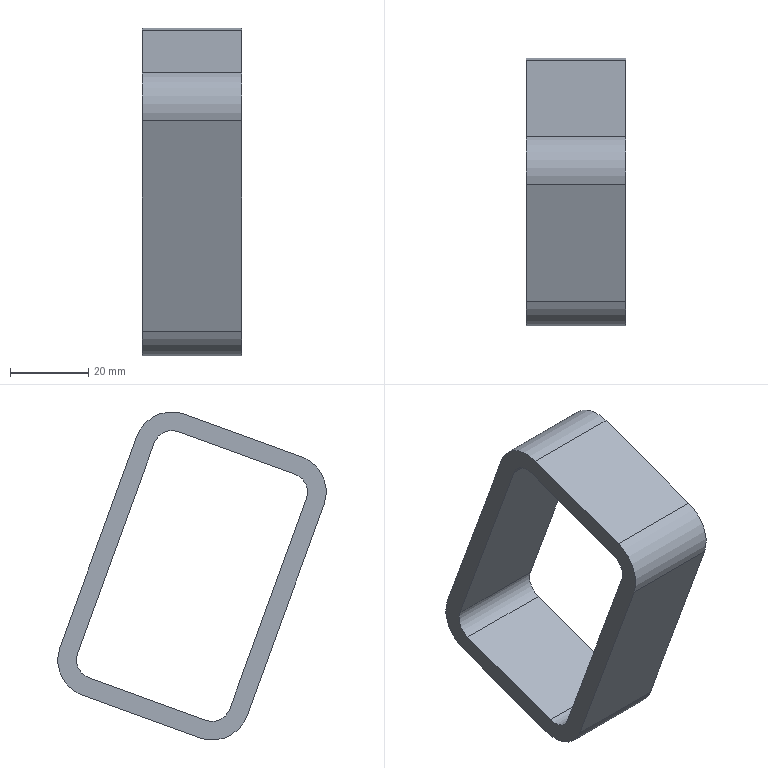Component | SolidWorks | rectangular tube_iso-69 | 1 solid | 18 faces | box 25.4 x 68.44 x 83.61 mm | volume 26938 mm3 | plane 10 | cylinder 8 | commonest cylinder face diameters 19.05 x4 9.525 x4
STEP:
#1=COLOUR_RGB('',0.7922,0.8196,0.9333);
#2=FILL_AREA_STYLE_COLOUR('',#1);
#3=FILL_AREA_STYLE('',(#2));
#4=SURFACE_STYLE_FILL_AREA(#3);
#5=SURFACE_SIDE_STYLE('',(#4));
#6=SURFACE_STYLE_USAGE(.BOTH.,#5);
#7=PRESENTATION_STYLE_ASSIGNMENT((#6));
#8=CARTESIAN_POINT('',(1.827,-40.871,5.613));
#9=VERTEX_POINT('',#8);
#10=CARTESIAN_POINT('',(1.827,-40.391,5.389));
#11=VERTEX_POINT('',#10);
#12=CARTESIAN_POINT('',(1.827,-40.519,5.741));
#13=DIRECTION('',(1.,-0.,0.));
#14=DIRECTION('',(0.,-0.9397,-0.3421));
#15=AXIS2_PLACEMENT_3D('',#12,#13,#14);
#16=CIRCLE('',#15,0.375);
#17=EDGE_CURVE('',#9,#11,#16,.T.);
#18=ORIENTED_EDGE('',*,*,#17,.T.);
#19=CARTESIAN_POINT('',(1.827,-39.216,5.817));
#20=VERTEX_POINT('',#19);
#21=CARTESIAN_POINT('',(1.827,-40.391,5.389));
#22=DIRECTION('',(0.,0.9397,0.3421));
#23=VECTOR('',#22,39.37);
#24=LINE('',#21,#23);
#25=EDGE_CURVE('',#11,#20,#24,.T.);
#26=ORIENTED_EDGE('',*,*,#25,.T.);
#27=CARTESIAN_POINT('',(1.827,-38.992,6.297));
#28=VERTEX_POINT('',#27);
#29=CARTESIAN_POINT('',(1.827,-39.344,6.169));
#30=DIRECTION('',(1.,-0.,0.));
#31=DIRECTION('',(0.,-0.9397,-0.3421));
#32=AXIS2_PLACEMENT_3D('',#29,#30,#31);
#33=CIRCLE('',#32,0.375);
#34=EDGE_CURVE('',#20,#28,#33,.T.);
#35=ORIENTED_EDGE('',*,*,#34,.T.);
#36=CARTESIAN_POINT('',(1.827,-39.762,8.412));
#37=VERTEX_POINT('',#36);
#38=CARTESIAN_POINT('',(1.827,-39.762,8.412));
#39=DIRECTION('',(-0.,-0.3421,0.9397));
#40=VECTOR('',#39,39.37);
#41=LINE('',#38,#40);
#42=EDGE_CURVE('',#28,#37,#41,.T.);
#43=ORIENTED_EDGE('',*,*,#42,.T.);
#44=CARTESIAN_POINT('',(1.827,-40.242,8.636));
#45=VERTEX_POINT('',#44);
#46=CARTESIAN_POINT('',(1.827,-40.114,8.283));
#47=DIRECTION('',(1.,-0.,0.));
#48=DIRECTION('',(0.,-0.9397,-0.3421));
#49=AXIS2_PLACEMENT_3D('',#46,#47,#48);
#50=CIRCLE('',#49,0.375);
#51=EDGE_CURVE('',#37,#45,#50,.T.);
#52=ORIENTED_EDGE('',*,*,#51,.T.);
#53=CARTESIAN_POINT('',(1.827,-41.417,8.208));
#54=VERTEX_POINT('',#53);
#55=CARTESIAN_POINT('',(1.827,-40.242,8.636));
#56=DIRECTION('',(-0.,-0.9397,-0.3421));
#57=VECTOR('',#56,39.37);
#58=LINE('',#55,#57);
#59=EDGE_CURVE('',#45,#54,#58,.T.);
#60=ORIENTED_EDGE('',*,*,#59,.T.);
#61=CARTESIAN_POINT('',(1.827,-41.641,7.727));
#62=VERTEX_POINT('',#61);
#63=CARTESIAN_POINT('',(1.827,-41.289,7.856));
#64=DIRECTION('',(1.,-0.,0.));
#65=DIRECTION('',(0.,-0.9397,-0.3421));
#66=AXIS2_PLACEMENT_3D('',#63,#64,#65);
#67=CIRCLE('',#66,0.375);
#68=EDGE_CURVE('',#54,#62,#67,.T.);
#69=ORIENTED_EDGE('',*,*,#68,.T.);
#70=CARTESIAN_POINT('',(1.827,-40.871,5.613));
#71=DIRECTION('',(0.,0.3421,-0.9397));
#72=VECTOR('',#71,39.37);
#73=LINE('',#70,#72);
#74=EDGE_CURVE('',#62,#9,#73,.T.);
#75=ORIENTED_EDGE('',*,*,#74,.T.);
#76=EDGE_LOOP('',(#18,#26,#35,#43,#52,#60,#69,#75));
#77=FACE_OUTER_BOUND('',#76,.T.);
#78=CARTESIAN_POINT('',(1.827,-39.168,6.233));
#79=VERTEX_POINT('',#78);
#80=CARTESIAN_POINT('',(1.827,-39.938,8.347));
#81=VERTEX_POINT('',#80);
#82=CARTESIAN_POINT('',(1.827,-39.938,8.347));
#83=DIRECTION('',(-0.,-0.3421,0.9397));
#84=VECTOR('',#83,39.37);
#85=LINE('',#82,#84);
#86=EDGE_CURVE('',#79,#81,#85,.T.);
#87=ORIENTED_EDGE('',*,*,#86,.F.);
#88=CARTESIAN_POINT('',(1.827,-39.28,5.993));
#89=VERTEX_POINT('',#88);
#90=CARTESIAN_POINT('',(1.827,-39.344,6.169));
#91=DIRECTION('',(1.,-0.,0.));
#92=DIRECTION('',(0.,-0.9397,-0.3421));
#93=AXIS2_PLACEMENT_3D('',#90,#91,#92);
#94=CIRCLE('',#93,0.1875);
#95=EDGE_CURVE('',#89,#79,#94,.T.);
#96=ORIENTED_EDGE('',*,*,#95,.F.);
#97=CARTESIAN_POINT('',(1.827,-40.455,5.565));
#98=VERTEX_POINT('',#97);
#99=CARTESIAN_POINT('',(1.827,-40.455,5.565));
#100=DIRECTION('',(0.,0.9397,0.3421));
#101=VECTOR('',#100,39.37);
#102=LINE('',#99,#101);
#103=EDGE_CURVE('',#98,#89,#102,.T.);
#104=ORIENTED_EDGE('',*,*,#103,.F.);
#105=CARTESIAN_POINT('',(1.827,-40.695,5.677));
#106=VERTEX_POINT('',#105);
#107=CARTESIAN_POINT('',(1.827,-40.519,5.741));
#108=DIRECTION('',(1.,-0.,0.));
#109=DIRECTION('',(0.,-0.9397,-0.3421));
#110=AXIS2_PLACEMENT_3D('',#107,#108,#109);
#111=CIRCLE('',#110,0.1875);
#112=EDGE_CURVE('',#106,#98,#111,.T.);
#113=ORIENTED_EDGE('',*,*,#112,.F.);
#114=CARTESIAN_POINT('',(1.827,-41.465,7.791));
#115=VERTEX_POINT('',#114);
#116=CARTESIAN_POINT('',(1.827,-40.695,5.677));
#117=DIRECTION('',(0.,0.3421,-0.9397));
#118=VECTOR('',#117,39.37);
#119=LINE('',#116,#118);
#120=EDGE_CURVE('',#115,#106,#119,.T.);
#121=ORIENTED_EDGE('',*,*,#120,.F.);
#122=CARTESIAN_POINT('',(1.827,-41.353,8.032));
#123=VERTEX_POINT('',#122);
#124=CARTESIAN_POINT('',(1.827,-41.289,7.856));
#125=DIRECTION('',(1.,-0.,0.));
#126=DIRECTION('',(0.,-0.9397,-0.3421));
#127=AXIS2_PLACEMENT_3D('',#124,#125,#126);
#128=CIRCLE('',#127,0.1875);
#129=EDGE_CURVE('',#123,#115,#128,.T.);
#130=ORIENTED_EDGE('',*,*,#129,.F.);
#131=CARTESIAN_POINT('',(1.827,-40.178,8.459));
#132=VERTEX_POINT('',#131);
#133=CARTESIAN_POINT('',(1.827,-40.178,8.459));
#134=DIRECTION('',(-0.,-0.9397,-0.3421));
#135=VECTOR('',#134,39.37);
#136=LINE('',#133,#135);
#137=EDGE_CURVE('',#132,#123,#136,.T.);
#138=ORIENTED_EDGE('',*,*,#137,.F.);
#139=CARTESIAN_POINT('',(1.827,-40.114,8.283));
#140=DIRECTION('',(1.,-0.,0.));
#141=DIRECTION('',(0.,-0.9397,-0.3421));
#142=AXIS2_PLACEMENT_3D('',#139,#140,#141);
#143=CIRCLE('',#142,0.1875);
#144=EDGE_CURVE('',#81,#132,#143,.T.);
#145=ORIENTED_EDGE('',*,*,#144,.F.);
#146=EDGE_LOOP('',(#87,#96,#104,#113,#121,#130,#138,#145));
#147=FACE_BOUND('',#146,.T.);
#148=CARTESIAN_POINT('',(1.827,-40.519,5.741));
#149=DIRECTION('',(1.,-0.,0.));
#150=DIRECTION('',(-0.,-0.9397,-0.3421));
#151=AXIS2_PLACEMENT_3D('',#148,#149,#150);
#152=PLANE('',#151);
#153=ADVANCED_FACE('',(#77,#147),#152,.T.);
#154=CARTESIAN_POINT('',(0.8268,-40.871,5.613));
#155=VERTEX_POINT('',#154);
#156=CARTESIAN_POINT('',(0.8268,-40.391,5.389));
#157=VERTEX_POINT('',#156);
#158=CARTESIAN_POINT('',(0.8268,-40.519,5.741));
#159=DIRECTION('',(1.,-0.,0.));
#160=DIRECTION('',(0.,-0.9397,-0.3421));
#161=AXIS2_PLACEMENT_3D('',#158,#159,#160);
#162=CIRCLE('',#161,0.375);
#163=EDGE_CURVE('',#155,#157,#162,.T.);
#164=ORIENTED_EDGE('',*,*,#163,.F.);
#165=CARTESIAN_POINT('',(0.8268,-41.641,7.727));
#166=VERTEX_POINT('',#165);
#167=CARTESIAN_POINT('',(0.8268,-40.871,5.613));
#168=DIRECTION('',(0.,0.3421,-0.9397));
#169=VECTOR('',#168,39.37);
#170=LINE('',#167,#169);
#171=EDGE_CURVE('',#166,#155,#170,.T.);
#172=ORIENTED_EDGE('',*,*,#171,.F.);
#173=CARTESIAN_POINT('',(0.8268,-41.417,8.208));
#174=VERTEX_POINT('',#173);
#175=CARTESIAN_POINT('',(0.8268,-41.289,7.856));
#176=DIRECTION('',(1.,-0.,0.));
#177=DIRECTION('',(0.,-0.9397,-0.3421));
#178=AXIS2_PLACEMENT_3D('',#175,#176,#177);
#179=CIRCLE('',#178,0.375);
#180=EDGE_CURVE('',#174,#166,#179,.T.);
#181=ORIENTED_EDGE('',*,*,#180,.F.);
#182=CARTESIAN_POINT('',(0.8268,-40.242,8.636));
#183=VERTEX_POINT('',#182);
#184=CARTESIAN_POINT('',(0.8268,-40.242,8.636));
#185=DIRECTION('',(-0.,-0.9397,-0.3421));
#186=VECTOR('',#185,39.37);
#187=LINE('',#184,#186);
#188=EDGE_CURVE('',#183,#174,#187,.T.);
#189=ORIENTED_EDGE('',*,*,#188,.F.);
#190=CARTESIAN_POINT('',(0.8268,-39.762,8.412));
#191=VERTEX_POINT('',#190);
#192=CARTESIAN_POINT('',(0.8268,-40.114,8.283));
#193=DIRECTION('',(1.,-0.,0.));
#194=DIRECTION('',(0.,-0.9397,-0.3421));
#195=AXIS2_PLACEMENT_3D('',#192,#193,#194);
#196=CIRCLE('',#195,0.375);
#197=EDGE_CURVE('',#191,#183,#196,.T.);
#198=ORIENTED_EDGE('',*,*,#197,.F.);
#199=CARTESIAN_POINT('',(0.8268,-38.992,6.297));
#200=VERTEX_POINT('',#199);
#201=CARTESIAN_POINT('',(0.8268,-39.762,8.412));
#202=DIRECTION('',(-0.,-0.3421,0.9397));
#203=VECTOR('',#202,39.37);
#204=LINE('',#201,#203);
#205=EDGE_CURVE('',#200,#191,#204,.T.);
#206=ORIENTED_EDGE('',*,*,#205,.F.);
#207=CARTESIAN_POINT('',(0.8268,-39.216,5.817));
#208=VERTEX_POINT('',#207);
#209=CARTESIAN_POINT('',(0.8268,-39.344,6.169));
#210=DIRECTION('',(1.,-0.,0.));
#211=DIRECTION('',(0.,-0.9397,-0.3421));
#212=AXIS2_PLACEMENT_3D('',#209,#210,#211);
#213=CIRCLE('',#212,0.375);
#214=EDGE_CURVE('',#208,#200,#213,.T.);
#215=ORIENTED_EDGE('',*,*,#214,.F.);
#216=CARTESIAN_POINT('',(0.8268,-40.391,5.389));
#217=DIRECTION('',(0.,0.9397,0.3421));
#218=VECTOR('',#217,39.37);
#219=LINE('',#216,#218);
#220=EDGE_CURVE('',#157,#208,#219,.T.);
#221=ORIENTED_EDGE('',*,*,#220,.F.);
#222=EDGE_LOOP('',(#164,#172,#181,#189,#198,#206,#215,#221));
#223=FACE_OUTER_BOUND('',#222,.T.);
#224=CARTESIAN_POINT('',(0.8268,-39.28,5.993));
#225=VERTEX_POINT('',#224);
#226=CARTESIAN_POINT('',(0.8268,-39.168,6.233));
#227=VERTEX_POINT('',#226);
#228=CARTESIAN_POINT('',(0.8268,-39.344,6.169));
#229=DIRECTION('',(1.,-0.,0.));
#230=DIRECTION('',(0.,-0.9397,-0.3421));
#231=AXIS2_PLACEMENT_3D('',#228,#229,#230);
#232=CIRCLE('',#231,0.1875);
#233=EDGE_CURVE('',#225,#227,#232,.T.);
#234=ORIENTED_EDGE('',*,*,#233,.T.);
#235=CARTESIAN_POINT('',(0.8268,-39.938,8.347));
#236=VERTEX_POINT('',#235);
#237=CARTESIAN_POINT('',(0.8268,-39.938,8.347));
#238=DIRECTION('',(-0.,-0.3421,0.9397));
#239=VECTOR('',#238,39.37);
#240=LINE('',#237,#239);
#241=EDGE_CURVE('',#227,#236,#240,.T.);
#242=ORIENTED_EDGE('',*,*,#241,.T.);
#243=CARTESIAN_POINT('',(0.8268,-40.178,8.459));
#244=VERTEX_POINT('',#243);
#245=CARTESIAN_POINT('',(0.8268,-40.114,8.283));
#246=DIRECTION('',(1.,-0.,0.));
#247=DIRECTION('',(0.,-0.9397,-0.3421));
#248=AXIS2_PLACEMENT_3D('',#245,#246,#247);
#249=CIRCLE('',#248,0.1875);
#250=EDGE_CURVE('',#236,#244,#249,.T.);
#251=ORIENTED_EDGE('',*,*,#250,.T.);
#252=CARTESIAN_POINT('',(0.8268,-41.353,8.032));
#253=VERTEX_POINT('',#252);
#254=CARTESIAN_POINT('',(0.8268,-40.178,8.459));
#255=DIRECTION('',(-0.,-0.9397,-0.3421));
#256=VECTOR('',#255,39.37);
#257=LINE('',#254,#256);
#258=EDGE_CURVE('',#244,#253,#257,.T.);
#259=ORIENTED_EDGE('',*,*,#258,.T.);
#260=CARTESIAN_POINT('',(0.8268,-41.465,7.791));
#261=VERTEX_POINT('',#260);
#262=CARTESIAN_POINT('',(0.8268,-41.289,7.856));
#263=DIRECTION('',(1.,-0.,0.));
#264=DIRECTION('',(0.,-0.9397,-0.3421));
#265=AXIS2_PLACEMENT_3D('',#262,#263,#264);
#266=CIRCLE('',#265,0.1875);
#267=EDGE_CURVE('',#253,#261,#266,.T.);
#268=ORIENTED_EDGE('',*,*,#267,.T.);
#269=CARTESIAN_POINT('',(0.8268,-40.695,5.677));
#270=VERTEX_POINT('',#269);
#271=CARTESIAN_POINT('',(0.8268,-40.695,5.677));
#272=DIRECTION('',(0.,0.3421,-0.9397));
#273=VECTOR('',#272,39.37);
#274=LINE('',#271,#273);
#275=EDGE_CURVE('',#261,#270,#274,.T.);
#276=ORIENTED_EDGE('',*,*,#275,.T.);
#277=CARTESIAN_POINT('',(0.8268,-40.455,5.565));
#278=VERTEX_POINT('',#277);
#279=CARTESIAN_POINT('',(0.8268,-40.519,5.741));
#280=DIRECTION('',(1.,-0.,0.));
#281=DIRECTION('',(0.,-0.9397,-0.3421));
#282=AXIS2_PLACEMENT_3D('',#279,#280,#281);
#283=CIRCLE('',#282,0.1875);
#284=EDGE_CURVE('',#270,#278,#283,.T.);
#285=ORIENTED_EDGE('',*,*,#284,.T.);
#286=CARTESIAN_POINT('',(0.8268,-40.455,5.565));
#287=DIRECTION('',(0.,0.9397,0.3421));
#288=VECTOR('',#287,39.37);
#289=LINE('',#286,#288);
#290=EDGE_CURVE('',#278,#225,#289,.T.);
#291=ORIENTED_EDGE('',*,*,#290,.T.);
#292=EDGE_LOOP('',(#234,#242,#251,#259,#268,#276,#285,#291));
#293=FACE_BOUND('',#292,.T.);
#294=CARTESIAN_POINT('',(0.8268,-40.519,5.741));
#295=DIRECTION('',(1.,-0.,0.));
#296=DIRECTION('',(-0.,-0.9397,-0.3421));
#297=AXIS2_PLACEMENT_3D('',#294,#295,#296);
#298=PLANE('',#297);
#299=ADVANCED_FACE('',(#223,#293),#298,.F.);
#300=ORIENTED_EDGE('',*,*,#163,.T.);
#301=CARTESIAN_POINT('',(1.827,-40.391,5.389));
#302=DIRECTION('',(-1.,0.,-0.));
#303=VECTOR('',#302,39.37);
#304=LINE('',#301,#303);
#305=EDGE_CURVE('',#11,#157,#304,.T.);
#306=ORIENTED_EDGE('',*,*,#305,.F.);
#307=ORIENTED_EDGE('',*,*,#17,.F.);
#308=CARTESIAN_POINT('',(1.827,-40.871,5.613));
#309=DIRECTION('',(-1.,0.,-0.));
#310=VECTOR('',#309,39.37);
#311=LINE('',#308,#310);
#312=EDGE_CURVE('',#9,#155,#311,.T.);
#313=ORIENTED_EDGE('',*,*,#312,.T.);
#314=EDGE_LOOP('',(#300,#306,#307,#313));
#315=FACE_OUTER_BOUND('',#314,.T.);
#316=CARTESIAN_POINT('',(1.827,-40.519,5.741));
#317=DIRECTION('',(-1.,0.,-0.));
#318=DIRECTION('',(0.,0.9397,0.3421));
#319=AXIS2_PLACEMENT_3D('',#316,#317,#318);
#320=CYLINDRICAL_SURFACE('',#319,0.375);
#321=ADVANCED_FACE('',(#315),#320,.T.);
#322=ORIENTED_EDGE('',*,*,#220,.T.);
#323=CARTESIAN_POINT('',(1.827,-39.216,5.817));
#324=DIRECTION('',(-1.,0.,-0.));
#325=VECTOR('',#324,39.37);
#326=LINE('',#323,#325);
#327=EDGE_CURVE('',#20,#208,#326,.T.);
#328=ORIENTED_EDGE('',*,*,#327,.F.);
#329=ORIENTED_EDGE('',*,*,#25,.F.);
#330=ORIENTED_EDGE('',*,*,#305,.T.);
#331=EDGE_LOOP('',(#322,#328,#329,#330));
#332=FACE_OUTER_BOUND('',#331,.T.);
#333=CARTESIAN_POINT('',(1.827,-40.391,5.389));
#334=DIRECTION('',(-0.,-0.3421,0.9397));
#335=DIRECTION('',(-0.,-0.9397,-0.3421));
#336=AXIS2_PLACEMENT_3D('',#333,#334,#335);
#337=PLANE('',#336);
#338=ADVANCED_FACE('',(#332),#337,.F.);
#339=ORIENTED_EDGE('',*,*,#214,.T.);
#340=CARTESIAN_POINT('',(1.827,-38.992,6.297));
#341=DIRECTION('',(-1.,0.,-0.));
#342=VECTOR('',#341,39.37);
#343=LINE('',#340,#342);
#344=EDGE_CURVE('',#28,#200,#343,.T.);
#345=ORIENTED_EDGE('',*,*,#344,.F.);
#346=ORIENTED_EDGE('',*,*,#34,.F.);
#347=ORIENTED_EDGE('',*,*,#327,.T.);
#348=EDGE_LOOP('',(#339,#345,#346,#347));
#349=FACE_OUTER_BOUND('',#348,.T.);
#350=CARTESIAN_POINT('',(1.827,-39.344,6.169));
#351=DIRECTION('',(-1.,0.,-0.));
#352=DIRECTION('',(0.,0.9397,0.3421));
#353=AXIS2_PLACEMENT_3D('',#350,#351,#352);
#354=CYLINDRICAL_SURFACE('',#353,0.375);
#355=ADVANCED_FACE('',(#349),#354,.T.);
#356=ORIENTED_EDGE('',*,*,#205,.T.);
#357=CARTESIAN_POINT('',(1.827,-39.762,8.412));
#358=DIRECTION('',(-1.,0.,-0.));
#359=VECTOR('',#358,39.37);
#360=LINE('',#357,#359);
#361=EDGE_CURVE('',#37,#191,#360,.T.);
#362=ORIENTED_EDGE('',*,*,#361,.F.);
#363=ORIENTED_EDGE('',*,*,#42,.F.);
#364=ORIENTED_EDGE('',*,*,#344,.T.);
#365=EDGE_LOOP('',(#356,#362,#363,#364));
#366=FACE_OUTER_BOUND('',#365,.T.);
#367=CARTESIAN_POINT('',(1.827,-39.762,8.412));
#368=DIRECTION('',(-0.,-0.9397,-0.3421));
#369=DIRECTION('',(0.,0.3421,-0.9397));
#370=AXIS2_PLACEMENT_3D('',#367,#368,#369);
#371=PLANE('',#370);
#372=ADVANCED_FACE('',(#366),#371,.F.);
#373=ORIENTED_EDGE('',*,*,#197,.T.);
#374=CARTESIAN_POINT('',(1.827,-40.242,8.636));
#375=DIRECTION('',(-1.,0.,-0.));
#376=VECTOR('',#375,39.37);
#377=LINE('',#374,#376);
#378=EDGE_CURVE('',#45,#183,#377,.T.);
#379=ORIENTED_EDGE('',*,*,#378,.F.);
#380=ORIENTED_EDGE('',*,*,#51,.F.);
#381=ORIENTED_EDGE('',*,*,#361,.T.);
#382=EDGE_LOOP('',(#373,#379,#380,#381));
#383=FACE_OUTER_BOUND('',#382,.T.);
#384=CARTESIAN_POINT('',(1.827,-40.114,8.283));
#385=DIRECTION('',(-1.,0.,-0.));
#386=DIRECTION('',(0.,0.9397,0.3421));
#387=AXIS2_PLACEMENT_3D('',#384,#385,#386);
#388=CYLINDRICAL_SURFACE('',#387,0.375);
#389=ADVANCED_FACE('',(#383),#388,.T.);
#390=ORIENTED_EDGE('',*,*,#188,.T.);
#391=CARTESIAN_POINT('',(1.827,-41.417,8.208));
#392=DIRECTION('',(-1.,0.,-0.));
#393=VECTOR('',#392,39.37);
#394=LINE('',#391,#393);
#395=EDGE_CURVE('',#54,#174,#394,.T.);
#396=ORIENTED_EDGE('',*,*,#395,.F.);
#397=ORIENTED_EDGE('',*,*,#59,.F.);
#398=ORIENTED_EDGE('',*,*,#378,.T.);
#399=EDGE_LOOP('',(#390,#396,#397,#398));
#400=FACE_OUTER_BOUND('',#399,.T.);
#401=CARTESIAN_POINT('',(1.827,-40.242,8.636));
#402=DIRECTION('',(0.,0.3421,-0.9397));
#403=DIRECTION('',(0.,0.9397,0.3421));
#404=AXIS2_PLACEMENT_3D('',#401,#402,#403);
#405=PLANE('',#404);
#406=ADVANCED_FACE('',(#400),#405,.F.);
#407=ORIENTED_EDGE('',*,*,#180,.T.);
#408=CARTESIAN_POINT('',(1.827,-41.641,7.727));
#409=DIRECTION('',(-1.,0.,-0.));
#410=VECTOR('',#409,39.37);
#411=LINE('',#408,#410);
#412=EDGE_CURVE('',#62,#166,#411,.T.);
#413=ORIENTED_EDGE('',*,*,#412,.F.);
#414=ORIENTED_EDGE('',*,*,#68,.F.);
#415=ORIENTED_EDGE('',*,*,#395,.T.);
#416=EDGE_LOOP('',(#407,#413,#414,#415));
#417=FACE_OUTER_BOUND('',#416,.T.);
#418=CARTESIAN_POINT('',(1.827,-41.289,7.856));
#419=DIRECTION('',(-1.,0.,-0.));
#420=DIRECTION('',(0.,0.9397,0.3421));
#421=AXIS2_PLACEMENT_3D('',#418,#419,#420);
#422=CYLINDRICAL_SURFACE('',#421,0.375);
#423=ADVANCED_FACE('',(#417),#422,.T.);
#424=ORIENTED_EDGE('',*,*,#171,.T.);
#425=ORIENTED_EDGE('',*,*,#312,.F.);
#426=ORIENTED_EDGE('',*,*,#74,.F.);
#427=ORIENTED_EDGE('',*,*,#412,.T.);
#428=EDGE_LOOP('',(#424,#425,#426,#427));
#429=FACE_OUTER_BOUND('',#428,.T.);
#430=CARTESIAN_POINT('',(1.827,-40.871,5.613));
#431=DIRECTION('',(0.,0.9397,0.3421));
#432=DIRECTION('',(-0.,-0.3421,0.9397));
#433=AXIS2_PLACEMENT_3D('',#430,#431,#432);
#434=PLANE('',#433);
#435=ADVANCED_FACE('',(#429),#434,.F.);
#436=ORIENTED_EDGE('',*,*,#233,.F.);
#437=CARTESIAN_POINT('',(1.827,-39.28,5.993));
#438=DIRECTION('',(-1.,0.,-0.));
#439=VECTOR('',#438,39.37);
#440=LINE('',#437,#439);
#441=EDGE_CURVE('',#89,#225,#440,.T.);
#442=ORIENTED_EDGE('',*,*,#441,.F.);
#443=ORIENTED_EDGE('',*,*,#95,.T.);
#444=CARTESIAN_POINT('',(1.827,-39.168,6.233));
#445=DIRECTION('',(-1.,0.,-0.));
#446=VECTOR('',#445,39.37);
#447=LINE('',#444,#446);
#448=EDGE_CURVE('',#79,#227,#447,.T.);
#449=ORIENTED_EDGE('',*,*,#448,.T.);
#450=EDGE_LOOP('',(#436,#442,#443,#449));
#451=FACE_OUTER_BOUND('',#450,.T.);
#452=CARTESIAN_POINT('',(1.827,-39.344,6.169));
#453=DIRECTION('',(-1.,0.,-0.));
#454=DIRECTION('',(0.,0.9397,0.3421));
#455=AXIS2_PLACEMENT_3D('',#452,#453,#454);
#456=CYLINDRICAL_SURFACE('',#455,0.1875);
#457=ADVANCED_FACE('',(#451),#456,.F.);
#458=ORIENTED_EDGE('',*,*,#241,.F.);
#459=ORIENTED_EDGE('',*,*,#448,.F.);
#460=ORIENTED_EDGE('',*,*,#86,.T.);
#461=CARTESIAN_POINT('',(1.827,-39.938,8.347));
#462=DIRECTION('',(-1.,0.,-0.));
#463=VECTOR('',#462,39.37);
#464=LINE('',#461,#463);
#465=EDGE_CURVE('',#81,#236,#464,.T.);
#466=ORIENTED_EDGE('',*,*,#465,.T.);
#467=EDGE_LOOP('',(#458,#459,#460,#466));
#468=FACE_OUTER_BOUND('',#467,.T.);
#469=CARTESIAN_POINT('',(1.827,-39.938,8.347));
#470=DIRECTION('',(-0.,-0.9397,-0.3421));
#471=DIRECTION('',(-1.,0.,-0.));
#472=AXIS2_PLACEMENT_3D('',#469,#470,#471);
#473=PLANE('',#472);
#474=ADVANCED_FACE('',(#468),#473,.T.);
#475=ORIENTED_EDGE('',*,*,#250,.F.);
#476=ORIENTED_EDGE('',*,*,#465,.F.);
#477=ORIENTED_EDGE('',*,*,#144,.T.);
#478=CARTESIAN_POINT('',(1.827,-40.178,8.459));
#479=DIRECTION('',(-1.,0.,-0.));
#480=VECTOR('',#479,39.37);
#481=LINE('',#478,#480);
#482=EDGE_CURVE('',#132,#244,#481,.T.);
#483=ORIENTED_EDGE('',*,*,#482,.T.);
#484=EDGE_LOOP('',(#475,#476,#477,#483));
#485=FACE_OUTER_BOUND('',#484,.T.);
#486=CARTESIAN_POINT('',(1.827,-40.114,8.283));
#487=DIRECTION('',(-1.,0.,-0.));
#488=DIRECTION('',(0.,0.9397,0.3421));
#489=AXIS2_PLACEMENT_3D('',#486,#487,#488);
#490=CYLINDRICAL_SURFACE('',#489,0.1875);
#491=ADVANCED_FACE('',(#485),#490,.F.);
#492=ORIENTED_EDGE('',*,*,#258,.F.);
#493=ORIENTED_EDGE('',*,*,#482,.F.);
#494=ORIENTED_EDGE('',*,*,#137,.T.);
#495=CARTESIAN_POINT('',(1.827,-41.353,8.032));
#496=DIRECTION('',(-1.,0.,-0.));
#497=VECTOR('',#496,39.37);
#498=LINE('',#495,#497);
#499=EDGE_CURVE('',#123,#253,#498,.T.);
#500=ORIENTED_EDGE('',*,*,#499,.T.);
#501=EDGE_LOOP('',(#492,#493,#494,#500));
#502=FACE_OUTER_BOUND('',#501,.T.);
#503=CARTESIAN_POINT('',(1.827,-40.178,8.459));
#504=DIRECTION('',(0.,0.3421,-0.9397));
#505=DIRECTION('',(0.,0.9397,0.3421));
#506=AXIS2_PLACEMENT_3D('',#503,#504,#505);
#507=PLANE('',#506);
#508=ADVANCED_FACE('',(#502),#507,.T.);
#509=ORIENTED_EDGE('',*,*,#267,.F.);
#510=ORIENTED_EDGE('',*,*,#499,.F.);
#511=ORIENTED_EDGE('',*,*,#129,.T.);
#512=CARTESIAN_POINT('',(1.827,-41.465,7.791));
#513=DIRECTION('',(-1.,0.,-0.));
#514=VECTOR('',#513,39.37);
#515=LINE('',#512,#514);
#516=EDGE_CURVE('',#115,#261,#515,.T.);
#517=ORIENTED_EDGE('',*,*,#516,.T.);
#518=EDGE_LOOP('',(#509,#510,#511,#517));
#519=FACE_OUTER_BOUND('',#518,.T.);
#520=CARTESIAN_POINT('',(1.827,-41.289,7.856));
#521=DIRECTION('',(-1.,0.,-0.));
#522=DIRECTION('',(0.,0.9397,0.3421));
#523=AXIS2_PLACEMENT_3D('',#520,#521,#522);
#524=CYLINDRICAL_SURFACE('',#523,0.1875);
#525=ADVANCED_FACE('',(#519),#524,.F.);
#526=ORIENTED_EDGE('',*,*,#275,.F.);
#527=ORIENTED_EDGE('',*,*,#516,.F.);
#528=ORIENTED_EDGE('',*,*,#120,.T.);
#529=CARTESIAN_POINT('',(1.827,-40.695,5.677));
#530=DIRECTION('',(-1.,0.,-0.));
#531=VECTOR('',#530,39.37);
#532=LINE('',#529,#531);
#533=EDGE_CURVE('',#106,#270,#532,.T.);
#534=ORIENTED_EDGE('',*,*,#533,.T.);
#535=EDGE_LOOP('',(#526,#527,#528,#534));
#536=FACE_OUTER_BOUND('',#535,.T.);
#537=CARTESIAN_POINT('',(1.827,-40.695,5.677));
#538=DIRECTION('',(0.,0.9397,0.3421));
#539=DIRECTION('',(-0.,-0.3421,0.9397));
#540=AXIS2_PLACEMENT_3D('',#537,#538,#539);
#541=PLANE('',#540);
#542=ADVANCED_FACE('',(#536),#541,.T.);
#543=ORIENTED_EDGE('',*,*,#284,.F.);
#544=ORIENTED_EDGE('',*,*,#533,.F.);
#545=ORIENTED_EDGE('',*,*,#112,.T.);
#546=CARTESIAN_POINT('',(1.827,-40.455,5.565));
#547=DIRECTION('',(-1.,0.,-0.));
#548=VECTOR('',#547,39.37);
#549=LINE('',#546,#548);
#550=EDGE_CURVE('',#98,#278,#549,.T.);
#551=ORIENTED_EDGE('',*,*,#550,.T.);
#552=EDGE_LOOP('',(#543,#544,#545,#551));
#553=FACE_OUTER_BOUND('',#552,.T.);
#554=CARTESIAN_POINT('',(1.827,-40.519,5.741));
#555=DIRECTION('',(-1.,0.,-0.));
#556=DIRECTION('',(0.,0.9397,0.3421));
#557=AXIS2_PLACEMENT_3D('',#554,#555,#556);
#558=CYLINDRICAL_SURFACE('',#557,0.1875);
#559=ADVANCED_FACE('',(#553),#558,.F.);
#560=ORIENTED_EDGE('',*,*,#290,.F.);
#561=ORIENTED_EDGE('',*,*,#550,.F.);
#562=ORIENTED_EDGE('',*,*,#103,.T.);
#563=ORIENTED_EDGE('',*,*,#441,.T.);
#564=EDGE_LOOP('',(#560,#561,#562,#563));
#565=FACE_OUTER_BOUND('',#564,.T.);
#566=CARTESIAN_POINT('',(1.827,-40.455,5.565));
#567=DIRECTION('',(-0.,-0.3421,0.9397));
#568=DIRECTION('',(-0.,-0.9397,-0.3421));
#569=AXIS2_PLACEMENT_3D('',#566,#567,#568);
#570=PLANE('',#569);
#571=ADVANCED_FACE('',(#565),#570,.T.);
#572=CLOSED_SHELL('',(#153,#299,#321,#338,#355,#372,#389,#406,#423,#435,#457,#474,#491,#508,#525,#542,#559,#571));
#573=MANIFOLD_SOLID_BREP('',#572);
#574=STYLED_ITEM('',(#7),#573);
#575=(LENGTH_UNIT()NAMED_UNIT(*)SI_UNIT($,.METRE.));
#576=LENGTH_MEASURE_WITH_UNIT(LENGTH_MEASURE(0.0254),#575);
#577=DIMENSIONAL_EXPONENTS(1.,0.,0.,0.,0.,0.,0.);
#578=(CONVERSION_BASED_UNIT('',#576)LENGTH_UNIT()NAMED_UNIT(#577));
#579=UNCERTAINTY_MEASURE_WITH_UNIT(LENGTH_MEASURE(0.00001),#578,'','');
#580=(NAMED_UNIT(*)PLANE_ANGLE_UNIT()SI_UNIT($,.RADIAN.));
#581=(NAMED_UNIT(*)SI_UNIT($,.STERADIAN.)SOLID_ANGLE_UNIT());
#582=(GEOMETRIC_REPRESENTATION_CONTEXT(3)GLOBAL_UNCERTAINTY_ASSIGNED_CONTEXT((#579))GLOBAL_UNIT_ASSIGNED_CONTEXT((#578,#580,#581))REPRESENTATION_CONTEXT('',''));
#583=MECHANICAL_DESIGN_GEOMETRIC_PRESENTATION_REPRESENTATION('',(#574),#582);
#584=CARTESIAN_POINT('',(0.,0.,0.));
#585=DIRECTION('',(0.,0.,1.));
#586=DIRECTION('',(1.,0.,0.));
#587=AXIS2_PLACEMENT_3D('',#584,#585,#586);
#588=(LENGTH_UNIT()NAMED_UNIT(*)SI_UNIT($,.METRE.));
#589=LENGTH_MEASURE_WITH_UNIT(LENGTH_MEASURE(0.0254),#588);
#590=DIMENSIONAL_EXPONENTS(1.,0.,0.,0.,0.,0.,0.);
#591=(CONVERSION_BASED_UNIT('',#589)LENGTH_UNIT()NAMED_UNIT(#590));
#592=UNCERTAINTY_MEASURE_WITH_UNIT(LENGTH_MEASURE(0.00001),#591,'','');
#593=(NAMED_UNIT(*)PLANE_ANGLE_UNIT()SI_UNIT($,.RADIAN.));
#594=(NAMED_UNIT(*)SI_UNIT($,.STERADIAN.)SOLID_ANGLE_UNIT());
#595=(GEOMETRIC_REPRESENTATION_CONTEXT(3)GLOBAL_UNCERTAINTY_ASSIGNED_CONTEXT((#592))GLOBAL_UNIT_ASSIGNED_CONTEXT((#591,#593,#594))REPRESENTATION_CONTEXT('',''));
#596=ADVANCED_BREP_SHAPE_REPRESENTATION('',(#573,#587),#595);
#597=PRESENTATION_LAYER_ASSIGNMENT('','',(#574));